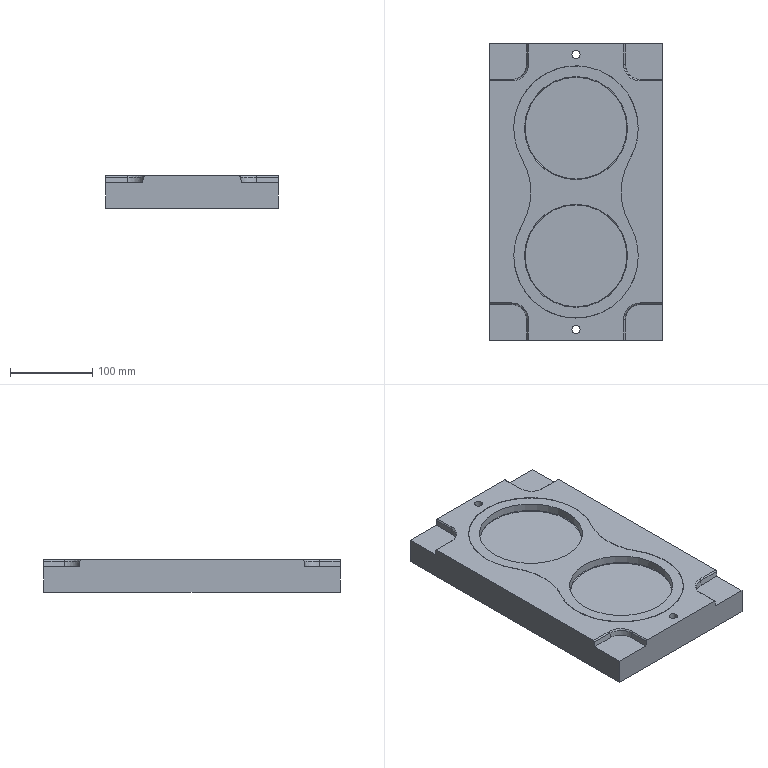CAM job | NX | mm | 3-axis | 1 set-up | 1 operations | part box 210 x 360 x 40
set-up 1
1. Cavity Milling | Mill Mill5 D17R0.8 | CAVITY_MILL | path 81795.344 mm | 314.369 min